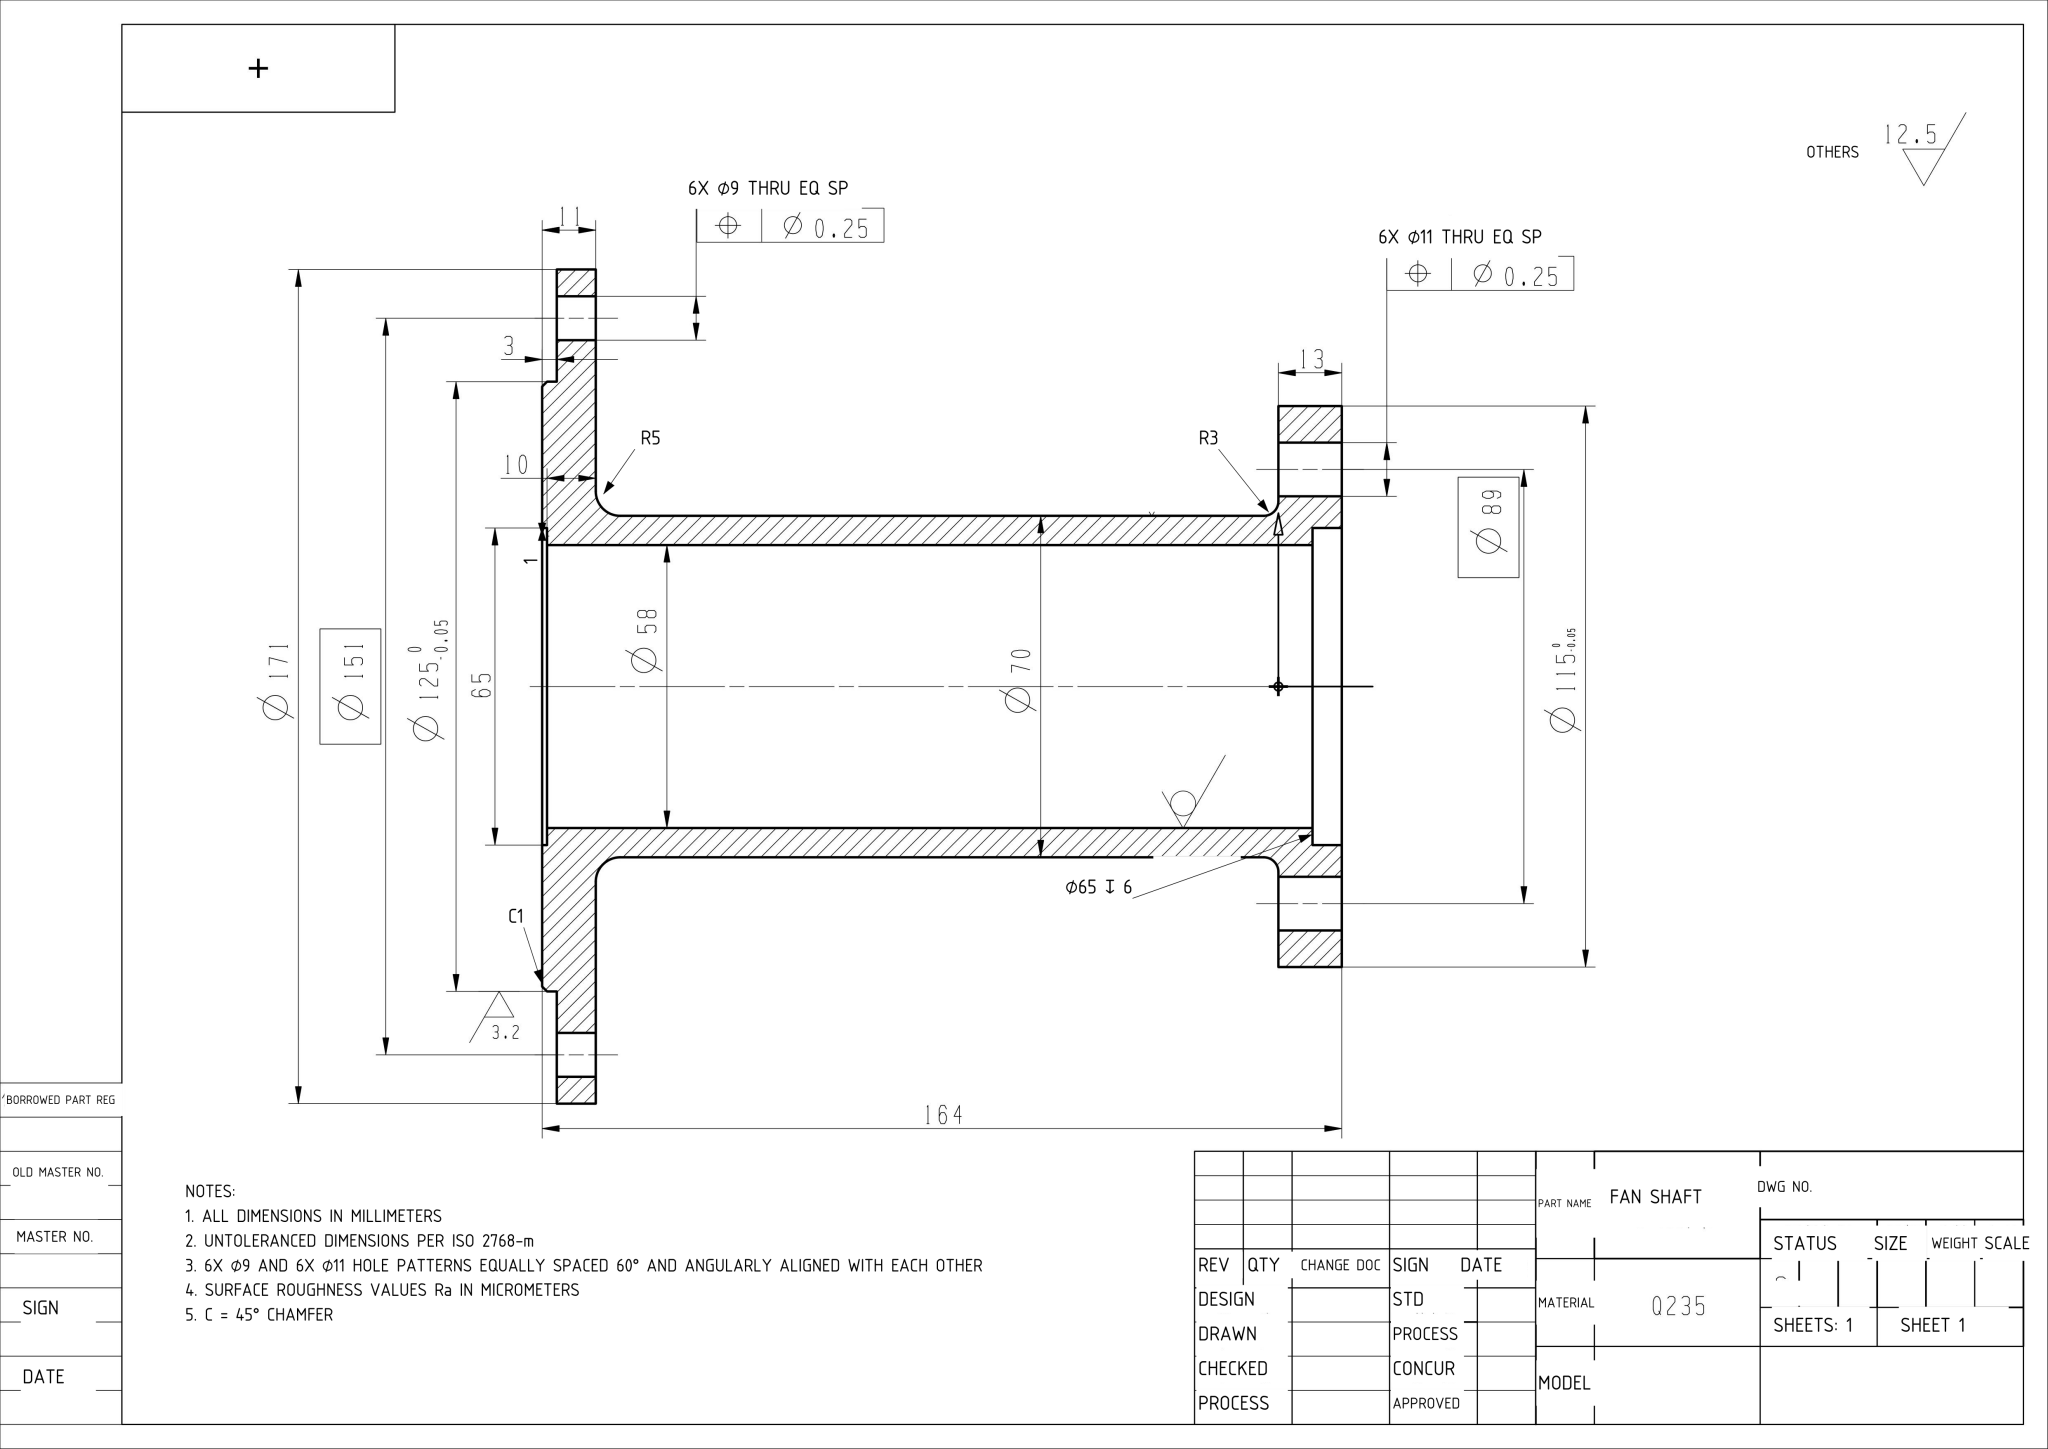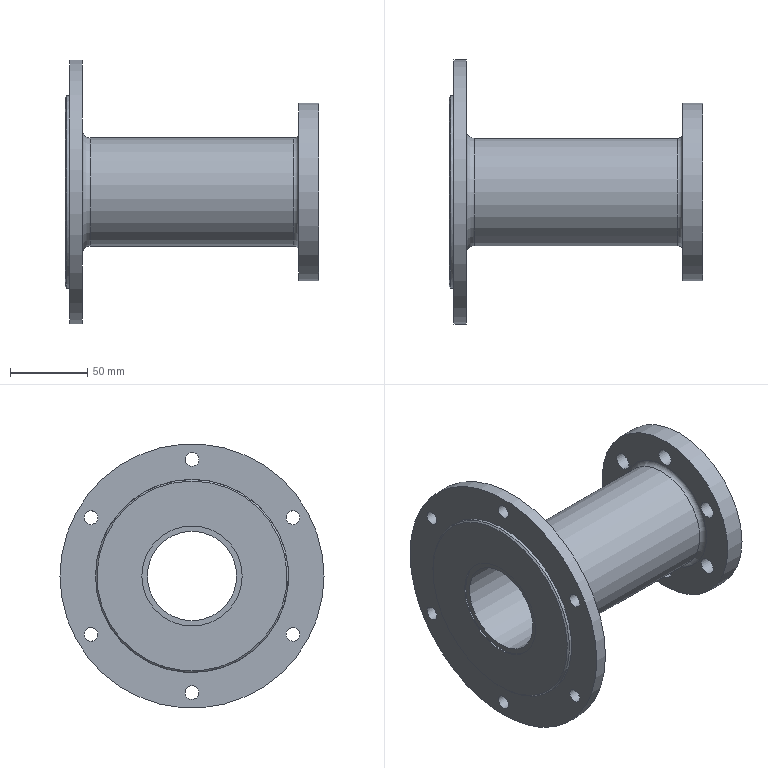Part | NX | mm | 1 solid | 29 faces | box 164 x 171 x 171 mm | volume 447309 mm3 | cylinder 19 | plane 7 | torus 2 | cone 1 | commonest cylinder face diameters 11 x6 9 x6 65 x2 70 x1 58 x1 115 x1 171 x1 125 x1
STEP:
#1=CARTESIAN_POINT('',(0.,0.,0.));
#2=DIRECTION('',(0.,0.,1.));
#3=DIRECTION('',(1.,0.,0.));
#4=AXIS2_PLACEMENT_3D('',#1,#2,#3);
#5=(LENGTH_UNIT()NAMED_UNIT(*)SI_UNIT(.MILLI.,.METRE.));
#6=UNCERTAINTY_MEASURE_WITH_UNIT(LENGTH_MEASURE(0.00002),#5,'','');
#7=(NAMED_UNIT(*)PLANE_ANGLE_UNIT()SI_UNIT($,.RADIAN.));
#8=PLANE_ANGLE_MEASURE_WITH_UNIT(PLANE_ANGLE_MEASURE(0.01745),#7);
#9=DIMENSIONAL_EXPONENTS(0.,0.,0.,0.,0.,0.,0.);
#10=(CONVERSION_BASED_UNIT('',#8)NAMED_UNIT(#9)PLANE_ANGLE_UNIT());
#11=(NAMED_UNIT(*)SI_UNIT($,.STERADIAN.)SOLID_ANGLE_UNIT());
#12=(GEOMETRIC_REPRESENTATION_CONTEXT(3)GLOBAL_UNCERTAINTY_ASSIGNED_CONTEXT((#6))GLOBAL_UNIT_ASSIGNED_CONTEXT((#5,#10,#11))REPRESENTATION_CONTEXT('',''));
#13=SHAPE_REPRESENTATION('',(#4),#12);
#14=CARTESIAN_POINT('',(-135.,0.,35.));
#15=VERTEX_POINT('',#14);
#16=CARTESIAN_POINT('',(-135.,0.,0.));
#17=DIRECTION('',(1.,0.,0.));
#18=DIRECTION('',(0.,0.,1.));
#19=AXIS2_PLACEMENT_3D('',#16,#17,#18);
#20=CIRCLE('',#19,35.);
#21=EDGE_CURVE('',#15,#15,#20,.T.);
#22=ORIENTED_EDGE('',*,*,#21,.T.);
#23=EDGE_LOOP('',(#22));
#24=FACE_BOUND('',#23,.T.);
#25=CARTESIAN_POINT('',(-3.,0.,-35.));
#26=VERTEX_POINT('',#25);
#27=CARTESIAN_POINT('',(-3.,0.,0.));
#28=DIRECTION('',(-1.,0.,0.));
#29=DIRECTION('',(0.,0.,-1.));
#30=AXIS2_PLACEMENT_3D('',#27,#28,#29);
#31=CIRCLE('',#30,35.);
#32=EDGE_CURVE('',#26,#26,#31,.T.);
#33=ORIENTED_EDGE('',*,*,#32,.T.);
#34=EDGE_LOOP('',(#33));
#35=FACE_BOUND('',#34,.T.);
#36=CARTESIAN_POINT('',(-140.,0.,0.));
#37=DIRECTION('',(1.,0.,0.));
#38=DIRECTION('',(0.,0.,-1.));
#39=AXIS2_PLACEMENT_3D('',#36,#37,#38);
#40=CYLINDRICAL_SURFACE('',#39,35.);
#41=ADVANCED_FACE('',(#24,#35),#40,.T.);
#42=CARTESIAN_POINT('',(-150.,0.,-29.));
#43=VERTEX_POINT('',#42);
#44=CARTESIAN_POINT('',(-150.,0.,0.));
#45=DIRECTION('',(-1.,0.,0.));
#46=DIRECTION('',(0.,0.,-1.));
#47=AXIS2_PLACEMENT_3D('',#44,#45,#46);
#48=CIRCLE('',#47,29.);
#49=EDGE_CURVE('',#43,#43,#48,.T.);
#50=ORIENTED_EDGE('',*,*,#49,.F.);
#51=EDGE_LOOP('',(#50));
#52=FACE_BOUND('',#51,.T.);
#53=CARTESIAN_POINT('',(-150.,32.5,-0.));
#54=VERTEX_POINT('',#53);
#55=CARTESIAN_POINT('',(-150.,0.,0.));
#56=DIRECTION('',(1.,0.,0.));
#57=DIRECTION('',(0.,1.,-0.));
#58=AXIS2_PLACEMENT_3D('',#55,#56,#57);
#59=CIRCLE('',#58,32.5);
#60=EDGE_CURVE('',#54,#54,#59,.T.);
#61=ORIENTED_EDGE('',*,*,#60,.F.);
#62=EDGE_LOOP('',(#61));
#63=FACE_BOUND('',#62,.T.);
#64=CARTESIAN_POINT('',(-150.,0.,0.));
#65=DIRECTION('',(1.,0.,0.));
#66=DIRECTION('',(0.,0.,-1.));
#67=AXIS2_PLACEMENT_3D('',#64,#65,#66);
#68=PLANE('',#67);
#69=ADVANCED_FACE('',(#52,#63),#68,.F.);
#70=CARTESIAN_POINT('',(7.,0.,-29.));
#71=VERTEX_POINT('',#70);
#72=CARTESIAN_POINT('',(7.,0.,0.));
#73=DIRECTION('',(-1.,0.,0.));
#74=DIRECTION('',(0.,0.,-1.));
#75=AXIS2_PLACEMENT_3D('',#72,#73,#74);
#76=CIRCLE('',#75,29.);
#77=EDGE_CURVE('',#71,#71,#76,.T.);
#78=ORIENTED_EDGE('',*,*,#77,.T.);
#79=EDGE_LOOP('',(#78));
#80=FACE_BOUND('',#79,.T.);
#81=CARTESIAN_POINT('',(7.,32.5,-0.));
#82=VERTEX_POINT('',#81);
#83=CARTESIAN_POINT('',(7.,0.,0.));
#84=DIRECTION('',(-1.,0.,0.));
#85=DIRECTION('',(0.,1.,-0.));
#86=AXIS2_PLACEMENT_3D('',#83,#84,#85);
#87=CIRCLE('',#86,32.5);
#88=EDGE_CURVE('',#82,#82,#87,.T.);
#89=ORIENTED_EDGE('',*,*,#88,.F.);
#90=EDGE_LOOP('',(#89));
#91=FACE_BOUND('',#90,.T.);
#92=CARTESIAN_POINT('',(7.,0.,0.));
#93=DIRECTION('',(1.,0.,0.));
#94=DIRECTION('',(0.,0.,-1.));
#95=AXIS2_PLACEMENT_3D('',#92,#93,#94);
#96=PLANE('',#95);
#97=ADVANCED_FACE('',(#80,#91),#96,.T.);
#98=ORIENTED_EDGE('',*,*,#77,.F.);
#99=EDGE_LOOP('',(#98));
#100=FACE_BOUND('',#99,.T.);
#101=ORIENTED_EDGE('',*,*,#49,.T.);
#102=EDGE_LOOP('',(#101));
#103=FACE_BOUND('',#102,.T.);
#104=CARTESIAN_POINT('',(-200.,0.,0.));
#105=DIRECTION('',(1.,0.,0.));
#106=DIRECTION('',(0.,0.,-1.));
#107=AXIS2_PLACEMENT_3D('',#104,#105,#106);
#108=CYLINDRICAL_SURFACE('',#107,29.);
#109=ADVANCED_FACE('',(#100,#103),#108,.F.);
#110=CARTESIAN_POINT('',(13.,0.,-32.5));
#111=VERTEX_POINT('',#110);
#112=CARTESIAN_POINT('',(13.,0.,0.));
#113=DIRECTION('',(1.,0.,0.));
#114=DIRECTION('',(0.,0.,-1.));
#115=AXIS2_PLACEMENT_3D('',#112,#113,#114);
#116=CIRCLE('',#115,32.5);
#117=EDGE_CURVE('',#111,#111,#116,.T.);
#118=ORIENTED_EDGE('',*,*,#117,.T.);
#119=EDGE_LOOP('',(#118));
#120=FACE_BOUND('',#119,.T.);
#121=ORIENTED_EDGE('',*,*,#88,.T.);
#122=EDGE_LOOP('',(#121));
#123=FACE_BOUND('',#122,.T.);
#124=CARTESIAN_POINT('',(20.,0.,0.));
#125=DIRECTION('',(-1.,0.,0.));
#126=DIRECTION('',(0.,0.,1.));
#127=AXIS2_PLACEMENT_3D('',#124,#125,#126);
#128=CYLINDRICAL_SURFACE('',#127,32.5);
#129=ADVANCED_FACE('',(#120,#123),#128,.F.);
#130=CARTESIAN_POINT('',(13.,57.5,-0.));
#131=VERTEX_POINT('',#130);
#132=CARTESIAN_POINT('',(13.,0.,0.));
#133=DIRECTION('',(1.,0.,0.));
#134=DIRECTION('',(0.,1.,-0.));
#135=AXIS2_PLACEMENT_3D('',#132,#133,#134);
#136=CIRCLE('',#135,57.5);
#137=EDGE_CURVE('',#131,#131,#136,.T.);
#138=ORIENTED_EDGE('',*,*,#137,.F.);
#139=EDGE_LOOP('',(#138));
#140=FACE_BOUND('',#139,.T.);
#141=CARTESIAN_POINT('',(0.,57.5,-0.));
#142=VERTEX_POINT('',#141);
#143=CARTESIAN_POINT('',(0.,0.,0.));
#144=DIRECTION('',(1.,0.,0.));
#145=DIRECTION('',(0.,1.,-0.));
#146=AXIS2_PLACEMENT_3D('',#143,#144,#145);
#147=CIRCLE('',#146,57.5);
#148=EDGE_CURVE('',#142,#142,#147,.T.);
#149=ORIENTED_EDGE('',*,*,#148,.T.);
#150=EDGE_LOOP('',(#149));
#151=FACE_BOUND('',#150,.T.);
#152=CARTESIAN_POINT('',(13.,0.,0.));
#153=DIRECTION('',(-1.,0.,0.));
#154=DIRECTION('',(0.,0.,1.));
#155=AXIS2_PLACEMENT_3D('',#152,#153,#154);
#156=CYLINDRICAL_SURFACE('',#155,57.5);
#157=ADVANCED_FACE('',(#140,#151),#156,.T.);
#158=CARTESIAN_POINT('',(13.,38.538,16.75));
#159=VERTEX_POINT('',#158);
#160=CARTESIAN_POINT('',(13.,38.538,22.25));
#161=DIRECTION('',(-1.,0.,0.));
#162=DIRECTION('',(0.,0.,-1.));
#163=AXIS2_PLACEMENT_3D('',#160,#161,#162);
#164=CIRCLE('',#163,5.5);
#165=EDGE_CURVE('',#159,#159,#164,.T.);
#166=ORIENTED_EDGE('',*,*,#165,.T.);
#167=EDGE_LOOP('',(#166));
#168=FACE_BOUND('',#167,.T.);
#169=CARTESIAN_POINT('',(13.,38.538,-27.75));
#170=VERTEX_POINT('',#169);
#171=CARTESIAN_POINT('',(13.,38.538,-22.25));
#172=DIRECTION('',(-1.,0.,0.));
#173=DIRECTION('',(0.,0.,-1.));
#174=AXIS2_PLACEMENT_3D('',#171,#172,#173);
#175=CIRCLE('',#174,5.5);
#176=EDGE_CURVE('',#170,#170,#175,.T.);
#177=ORIENTED_EDGE('',*,*,#176,.T.);
#178=EDGE_LOOP('',(#177));
#179=FACE_BOUND('',#178,.T.);
#180=CARTESIAN_POINT('',(13.,-0.,-50.));
#181=VERTEX_POINT('',#180);
#182=CARTESIAN_POINT('',(13.,-0.,-44.5));
#183=DIRECTION('',(-1.,0.,0.));
#184=DIRECTION('',(0.,0.,-1.));
#185=AXIS2_PLACEMENT_3D('',#182,#183,#184);
#186=CIRCLE('',#185,5.5);
#187=EDGE_CURVE('',#181,#181,#186,.T.);
#188=ORIENTED_EDGE('',*,*,#187,.T.);
#189=EDGE_LOOP('',(#188));
#190=FACE_BOUND('',#189,.T.);
#191=CARTESIAN_POINT('',(13.,-38.538,-27.75));
#192=VERTEX_POINT('',#191);
#193=CARTESIAN_POINT('',(13.,-38.538,-22.25));
#194=DIRECTION('',(-1.,0.,0.));
#195=DIRECTION('',(0.,0.,-1.));
#196=AXIS2_PLACEMENT_3D('',#193,#194,#195);
#197=CIRCLE('',#196,5.5);
#198=EDGE_CURVE('',#192,#192,#197,.T.);
#199=ORIENTED_EDGE('',*,*,#198,.T.);
#200=EDGE_LOOP('',(#199));
#201=FACE_BOUND('',#200,.T.);
#202=CARTESIAN_POINT('',(13.,-38.538,16.75));
#203=VERTEX_POINT('',#202);
#204=CARTESIAN_POINT('',(13.,-38.538,22.25));
#205=DIRECTION('',(-1.,0.,0.));
#206=DIRECTION('',(0.,0.,-1.));
#207=AXIS2_PLACEMENT_3D('',#204,#205,#206);
#208=CIRCLE('',#207,5.5);
#209=EDGE_CURVE('',#203,#203,#208,.T.);
#210=ORIENTED_EDGE('',*,*,#209,.T.);
#211=EDGE_LOOP('',(#210));
#212=FACE_BOUND('',#211,.T.);
#213=CARTESIAN_POINT('',(13.,0.,39.));
#214=VERTEX_POINT('',#213);
#215=CARTESIAN_POINT('',(13.,0.,44.5));
#216=DIRECTION('',(-1.,0.,0.));
#217=DIRECTION('',(0.,0.,-1.));
#218=AXIS2_PLACEMENT_3D('',#215,#216,#217);
#219=CIRCLE('',#218,5.5);
#220=EDGE_CURVE('',#214,#214,#219,.T.);
#221=ORIENTED_EDGE('',*,*,#220,.T.);
#222=EDGE_LOOP('',(#221));
#223=FACE_BOUND('',#222,.T.);
#224=ORIENTED_EDGE('',*,*,#117,.F.);
#225=EDGE_LOOP('',(#224));
#226=FACE_BOUND('',#225,.T.);
#227=ORIENTED_EDGE('',*,*,#137,.T.);
#228=EDGE_LOOP('',(#227));
#229=FACE_BOUND('',#228,.T.);
#230=CARTESIAN_POINT('',(13.,0.,0.));
#231=DIRECTION('',(1.,0.,0.));
#232=DIRECTION('',(0.,0.,-1.));
#233=AXIS2_PLACEMENT_3D('',#230,#231,#232);
#234=PLANE('',#233);
#235=ADVANCED_FACE('',(#168,#179,#190,#201,#212,#223,#226,#229),#234,.T.);
#236=CARTESIAN_POINT('',(0.,0.,-38.));
#237=VERTEX_POINT('',#236);
#238=CARTESIAN_POINT('',(0.,0.,0.));
#239=DIRECTION('',(1.,0.,0.));
#240=DIRECTION('',(0.,0.,-1.));
#241=AXIS2_PLACEMENT_3D('',#238,#239,#240);
#242=CIRCLE('',#241,38.);
#243=EDGE_CURVE('',#237,#237,#242,.T.);
#244=ORIENTED_EDGE('',*,*,#243,.T.);
#245=EDGE_LOOP('',(#244));
#246=FACE_BOUND('',#245,.T.);
#247=CARTESIAN_POINT('',(0.,41.288,17.487));
#248=VERTEX_POINT('',#247);
#249=CARTESIAN_POINT('',(0.,38.538,22.25));
#250=DIRECTION('',(1.,0.,0.));
#251=DIRECTION('',(0.,0.5,-0.866));
#252=AXIS2_PLACEMENT_3D('',#249,#250,#251);
#253=CIRCLE('',#252,5.5);
#254=EDGE_CURVE('',#248,#248,#253,.T.);
#255=ORIENTED_EDGE('',*,*,#254,.T.);
#256=EDGE_LOOP('',(#255));
#257=FACE_BOUND('',#256,.T.);
#258=CARTESIAN_POINT('',(0.,35.788,-27.013));
#259=VERTEX_POINT('',#258);
#260=CARTESIAN_POINT('',(0.,38.538,-22.25));
#261=DIRECTION('',(1.,0.,0.));
#262=DIRECTION('',(0.,-0.5,-0.866));
#263=AXIS2_PLACEMENT_3D('',#260,#261,#262);
#264=CIRCLE('',#263,5.5);
#265=EDGE_CURVE('',#259,#259,#264,.T.);
#266=ORIENTED_EDGE('',*,*,#265,.T.);
#267=EDGE_LOOP('',(#266));
#268=FACE_BOUND('',#267,.T.);
#269=CARTESIAN_POINT('',(0.,-5.5,-44.5));
#270=VERTEX_POINT('',#269);
#271=CARTESIAN_POINT('',(0.,-0.,-44.5));
#272=DIRECTION('',(1.,0.,0.));
#273=DIRECTION('',(0.,-1.,0.));
#274=AXIS2_PLACEMENT_3D('',#271,#272,#273);
#275=CIRCLE('',#274,5.5);
#276=EDGE_CURVE('',#270,#270,#275,.T.);
#277=ORIENTED_EDGE('',*,*,#276,.T.);
#278=EDGE_LOOP('',(#277));
#279=FACE_BOUND('',#278,.T.);
#280=CARTESIAN_POINT('',(0.,-41.288,-17.487));
#281=VERTEX_POINT('',#280);
#282=CARTESIAN_POINT('',(0.,-38.538,-22.25));
#283=DIRECTION('',(1.,0.,0.));
#284=DIRECTION('',(0.,-0.5,0.866));
#285=AXIS2_PLACEMENT_3D('',#282,#283,#284);
#286=CIRCLE('',#285,5.5);
#287=EDGE_CURVE('',#281,#281,#286,.T.);
#288=ORIENTED_EDGE('',*,*,#287,.T.);
#289=EDGE_LOOP('',(#288));
#290=FACE_BOUND('',#289,.T.);
#291=CARTESIAN_POINT('',(0.,-35.788,27.013));
#292=VERTEX_POINT('',#291);
#293=CARTESIAN_POINT('',(0.,-38.538,22.25));
#294=DIRECTION('',(1.,0.,0.));
#295=DIRECTION('',(0.,0.5,0.866));
#296=AXIS2_PLACEMENT_3D('',#293,#294,#295);
#297=CIRCLE('',#296,5.5);
#298=EDGE_CURVE('',#292,#292,#297,.T.);
#299=ORIENTED_EDGE('',*,*,#298,.T.);
#300=EDGE_LOOP('',(#299));
#301=FACE_BOUND('',#300,.T.);
#302=CARTESIAN_POINT('',(0.,5.5,44.5));
#303=VERTEX_POINT('',#302);
#304=CARTESIAN_POINT('',(0.,0.,44.5));
#305=DIRECTION('',(1.,0.,0.));
#306=DIRECTION('',(0.,1.,0.));
#307=AXIS2_PLACEMENT_3D('',#304,#305,#306);
#308=CIRCLE('',#307,5.5);
#309=EDGE_CURVE('',#303,#303,#308,.T.);
#310=ORIENTED_EDGE('',*,*,#309,.T.);
#311=EDGE_LOOP('',(#310));
#312=FACE_BOUND('',#311,.T.);
#313=ORIENTED_EDGE('',*,*,#148,.F.);
#314=EDGE_LOOP('',(#313));
#315=FACE_BOUND('',#314,.T.);
#316=CARTESIAN_POINT('',(0.,0.,0.));
#317=DIRECTION('',(1.,0.,0.));
#318=DIRECTION('',(0.,0.,-1.));
#319=AXIS2_PLACEMENT_3D('',#316,#317,#318);
#320=PLANE('',#319);
#321=ADVANCED_FACE('',(#246,#257,#268,#279,#290,#301,#312,#315),#320,.F.);
#322=ORIENTED_EDGE('',*,*,#220,.F.);
#323=EDGE_LOOP('',(#322));
#324=FACE_BOUND('',#323,.T.);
#325=ORIENTED_EDGE('',*,*,#309,.F.);
#326=EDGE_LOOP('',(#325));
#327=FACE_BOUND('',#326,.T.);
#328=CARTESIAN_POINT('',(20.,0.,44.5));
#329=DIRECTION('',(-1.,0.,0.));
#330=DIRECTION('',(0.,0.,1.));
#331=AXIS2_PLACEMENT_3D('',#328,#329,#330);
#332=CYLINDRICAL_SURFACE('',#331,5.5);
#333=ADVANCED_FACE('',(#324,#327),#332,.F.);
#334=ORIENTED_EDGE('',*,*,#209,.F.);
#335=EDGE_LOOP('',(#334));
#336=FACE_BOUND('',#335,.T.);
#337=ORIENTED_EDGE('',*,*,#298,.F.);
#338=EDGE_LOOP('',(#337));
#339=FACE_BOUND('',#338,.T.);
#340=CARTESIAN_POINT('',(20.,-38.538,22.25));
#341=DIRECTION('',(-1.,0.,0.));
#342=DIRECTION('',(0.,0.,1.));
#343=AXIS2_PLACEMENT_3D('',#340,#341,#342);
#344=CYLINDRICAL_SURFACE('',#343,5.5);
#345=ADVANCED_FACE('',(#336,#339),#344,.F.);
#346=ORIENTED_EDGE('',*,*,#198,.F.);
#347=EDGE_LOOP('',(#346));
#348=FACE_BOUND('',#347,.T.);
#349=ORIENTED_EDGE('',*,*,#287,.F.);
#350=EDGE_LOOP('',(#349));
#351=FACE_BOUND('',#350,.T.);
#352=CARTESIAN_POINT('',(20.,-38.538,-22.25));
#353=DIRECTION('',(-1.,0.,0.));
#354=DIRECTION('',(0.,0.,1.));
#355=AXIS2_PLACEMENT_3D('',#352,#353,#354);
#356=CYLINDRICAL_SURFACE('',#355,5.5);
#357=ADVANCED_FACE('',(#348,#351),#356,.F.);
#358=ORIENTED_EDGE('',*,*,#187,.F.);
#359=EDGE_LOOP('',(#358));
#360=FACE_BOUND('',#359,.T.);
#361=ORIENTED_EDGE('',*,*,#276,.F.);
#362=EDGE_LOOP('',(#361));
#363=FACE_BOUND('',#362,.T.);
#364=CARTESIAN_POINT('',(20.,-0.,-44.5));
#365=DIRECTION('',(-1.,0.,0.));
#366=DIRECTION('',(0.,0.,1.));
#367=AXIS2_PLACEMENT_3D('',#364,#365,#366);
#368=CYLINDRICAL_SURFACE('',#367,5.5);
#369=ADVANCED_FACE('',(#360,#363),#368,.F.);
#370=ORIENTED_EDGE('',*,*,#176,.F.);
#371=EDGE_LOOP('',(#370));
#372=FACE_BOUND('',#371,.T.);
#373=ORIENTED_EDGE('',*,*,#265,.F.);
#374=EDGE_LOOP('',(#373));
#375=FACE_BOUND('',#374,.T.);
#376=CARTESIAN_POINT('',(20.,38.538,-22.25));
#377=DIRECTION('',(-1.,0.,0.));
#378=DIRECTION('',(0.,0.,1.));
#379=AXIS2_PLACEMENT_3D('',#376,#377,#378);
#380=CYLINDRICAL_SURFACE('',#379,5.5);
#381=ADVANCED_FACE('',(#372,#375),#380,.F.);
#382=ORIENTED_EDGE('',*,*,#165,.F.);
#383=EDGE_LOOP('',(#382));
#384=FACE_BOUND('',#383,.T.);
#385=ORIENTED_EDGE('',*,*,#254,.F.);
#386=EDGE_LOOP('',(#385));
#387=FACE_BOUND('',#386,.T.);
#388=CARTESIAN_POINT('',(20.,38.538,22.25));
#389=DIRECTION('',(-1.,0.,0.));
#390=DIRECTION('',(0.,0.,1.));
#391=AXIS2_PLACEMENT_3D('',#388,#389,#390);
#392=CYLINDRICAL_SURFACE('',#391,5.5);
#393=ADVANCED_FACE('',(#384,#387),#392,.F.);
#394=CARTESIAN_POINT('',(-140.,0.,40.));
#395=VERTEX_POINT('',#394);
#396=CARTESIAN_POINT('',(-140.,0.,0.));
#397=DIRECTION('',(-1.,0.,0.));
#398=DIRECTION('',(0.,0.,1.));
#399=AXIS2_PLACEMENT_3D('',#396,#397,#398);
#400=CIRCLE('',#399,40.);
#401=EDGE_CURVE('',#395,#395,#400,.T.);
#402=ORIENTED_EDGE('',*,*,#401,.T.);
#403=EDGE_LOOP('',(#402));
#404=FACE_BOUND('',#403,.T.);
#405=CARTESIAN_POINT('',(-140.,85.5,0.));
#406=VERTEX_POINT('',#405);
#407=CARTESIAN_POINT('',(-140.,0.,0.));
#408=DIRECTION('',(-1.,0.,0.));
#409=DIRECTION('',(0.,1.,0.));
#410=AXIS2_PLACEMENT_3D('',#407,#408,#409);
#411=CIRCLE('',#410,85.5);
#412=EDGE_CURVE('',#406,#406,#411,.T.);
#413=ORIENTED_EDGE('',*,*,#412,.F.);
#414=EDGE_LOOP('',(#413));
#415=FACE_BOUND('',#414,.T.);
#416=CARTESIAN_POINT('',(-140.,4.5,-75.5));
#417=VERTEX_POINT('',#416);
#418=CARTESIAN_POINT('',(-140.,0.,-75.5));
#419=DIRECTION('',(1.,0.,0.));
#420=DIRECTION('',(0.,1.,0.));
#421=AXIS2_PLACEMENT_3D('',#418,#419,#420);
#422=CIRCLE('',#421,4.5);
#423=EDGE_CURVE('',#417,#417,#422,.T.);
#424=ORIENTED_EDGE('',*,*,#423,.F.);
#425=EDGE_LOOP('',(#424));
#426=FACE_BOUND('',#425,.T.);
#427=CARTESIAN_POINT('',(-140.,67.635,-33.853));
#428=VERTEX_POINT('',#427);
#429=CARTESIAN_POINT('',(-140.,65.385,-37.75));
#430=DIRECTION('',(1.,0.,0.));
#431=DIRECTION('',(0.,0.5,0.866));
#432=AXIS2_PLACEMENT_3D('',#429,#430,#431);
#433=CIRCLE('',#432,4.5);
#434=EDGE_CURVE('',#428,#428,#433,.T.);
#435=ORIENTED_EDGE('',*,*,#434,.F.);
#436=EDGE_LOOP('',(#435));
#437=FACE_BOUND('',#436,.T.);
#438=CARTESIAN_POINT('',(-140.,63.135,41.647));
#439=VERTEX_POINT('',#438);
#440=CARTESIAN_POINT('',(-140.,65.385,37.75));
#441=DIRECTION('',(1.,0.,0.));
#442=DIRECTION('',(0.,-0.5,0.866));
#443=AXIS2_PLACEMENT_3D('',#440,#441,#442);
#444=CIRCLE('',#443,4.5);
#445=EDGE_CURVE('',#439,#439,#444,.T.);
#446=ORIENTED_EDGE('',*,*,#445,.F.);
#447=EDGE_LOOP('',(#446));
#448=FACE_BOUND('',#447,.T.);
#449=CARTESIAN_POINT('',(-140.,-4.5,75.5));
#450=VERTEX_POINT('',#449);
#451=CARTESIAN_POINT('',(-140.,0.,75.5));
#452=DIRECTION('',(1.,0.,0.));
#453=DIRECTION('',(0.,-1.,0.));
#454=AXIS2_PLACEMENT_3D('',#451,#452,#453);
#455=CIRCLE('',#454,4.5);
#456=EDGE_CURVE('',#450,#450,#455,.T.);
#457=ORIENTED_EDGE('',*,*,#456,.F.);
#458=EDGE_LOOP('',(#457));
#459=FACE_BOUND('',#458,.T.);
#460=CARTESIAN_POINT('',(-140.,-67.635,33.853));
#461=VERTEX_POINT('',#460);
#462=CARTESIAN_POINT('',(-140.,-65.385,37.75));
#463=DIRECTION('',(1.,0.,0.));
#464=DIRECTION('',(0.,-0.5,-0.866));
#465=AXIS2_PLACEMENT_3D('',#462,#463,#464);
#466=CIRCLE('',#465,4.5);
#467=EDGE_CURVE('',#461,#461,#466,.T.);
#468=ORIENTED_EDGE('',*,*,#467,.F.);
#469=EDGE_LOOP('',(#468));
#470=FACE_BOUND('',#469,.T.);
#471=CARTESIAN_POINT('',(-140.,-63.135,-41.647));
#472=VERTEX_POINT('',#471);
#473=CARTESIAN_POINT('',(-140.,-65.385,-37.75));
#474=DIRECTION('',(1.,0.,0.));
#475=DIRECTION('',(0.,0.5,-0.866));
#476=AXIS2_PLACEMENT_3D('',#473,#474,#475);
#477=CIRCLE('',#476,4.5);
#478=EDGE_CURVE('',#472,#472,#477,.T.);
#479=ORIENTED_EDGE('',*,*,#478,.F.);
#480=EDGE_LOOP('',(#479));
#481=FACE_BOUND('',#480,.T.);
#482=CARTESIAN_POINT('',(-140.,0.,0.));
#483=DIRECTION('',(-1.,0.,0.));
#484=DIRECTION('',(0.,0.,1.));
#485=AXIS2_PLACEMENT_3D('',#482,#483,#484);
#486=PLANE('',#485);
#487=ADVANCED_FACE('',(#404,#415,#426,#437,#448,#459,#470,#481),#486,.F.);
#488=ORIENTED_EDGE('',*,*,#412,.T.);
#489=EDGE_LOOP('',(#488));
#490=FACE_BOUND('',#489,.T.);
#491=CARTESIAN_POINT('',(-148.,85.5,0.));
#492=VERTEX_POINT('',#491);
#493=CARTESIAN_POINT('',(-148.,0.,0.));
#494=DIRECTION('',(-1.,0.,0.));
#495=DIRECTION('',(0.,1.,0.));
#496=AXIS2_PLACEMENT_3D('',#493,#494,#495);
#497=CIRCLE('',#496,85.5);
#498=EDGE_CURVE('',#492,#492,#497,.T.);
#499=ORIENTED_EDGE('',*,*,#498,.F.);
#500=EDGE_LOOP('',(#499));
#501=FACE_BOUND('',#500,.T.);
#502=CARTESIAN_POINT('',(-151.,0.,0.));
#503=DIRECTION('',(1.,0.,0.));
#504=DIRECTION('',(0.,0.,-1.));
#505=AXIS2_PLACEMENT_3D('',#502,#503,#504);
#506=CYLINDRICAL_SURFACE('',#505,85.5);
#507=ADVANCED_FACE('',(#490,#501),#506,.T.);
#508=CARTESIAN_POINT('',(-151.,0.,61.5));
#509=VERTEX_POINT('',#508);
#510=CARTESIAN_POINT('',(-151.,0.,0.));
#511=DIRECTION('',(-1.,0.,0.));
#512=DIRECTION('',(0.,0.,1.));
#513=AXIS2_PLACEMENT_3D('',#510,#511,#512);
#514=CIRCLE('',#513,61.5);
#515=EDGE_CURVE('',#509,#509,#514,.T.);
#516=ORIENTED_EDGE('',*,*,#515,.T.);
#517=EDGE_LOOP('',(#516));
#518=FACE_BOUND('',#517,.T.);
#519=CARTESIAN_POINT('',(-151.,32.5,0.));
#520=VERTEX_POINT('',#519);
#521=CARTESIAN_POINT('',(-151.,0.,0.));
#522=DIRECTION('',(-1.,0.,0.));
#523=DIRECTION('',(0.,1.,0.));
#524=AXIS2_PLACEMENT_3D('',#521,#522,#523);
#525=CIRCLE('',#524,32.5);
#526=EDGE_CURVE('',#520,#520,#525,.T.);
#527=ORIENTED_EDGE('',*,*,#526,.F.);
#528=EDGE_LOOP('',(#527));
#529=FACE_BOUND('',#528,.T.);
#530=CARTESIAN_POINT('',(-151.,0.,0.));
#531=DIRECTION('',(-1.,0.,0.));
#532=DIRECTION('',(0.,0.,1.));
#533=AXIS2_PLACEMENT_3D('',#530,#531,#532);
#534=PLANE('',#533);
#535=ADVANCED_FACE('',(#518,#529),#534,.T.);
#536=ORIENTED_EDGE('',*,*,#60,.T.);
#537=EDGE_LOOP('',(#536));
#538=FACE_BOUND('',#537,.T.);
#539=ORIENTED_EDGE('',*,*,#526,.T.);
#540=EDGE_LOOP('',(#539));
#541=FACE_BOUND('',#540,.T.);
#542=CARTESIAN_POINT('',(-151.,0.,0.));
#543=DIRECTION('',(1.,0.,0.));
#544=DIRECTION('',(0.,0.,-1.));
#545=AXIS2_PLACEMENT_3D('',#542,#543,#544);
#546=CYLINDRICAL_SURFACE('',#545,32.5);
#547=ADVANCED_FACE('',(#538,#541),#546,.F.);
#548=CARTESIAN_POINT('',(-150.,0.,62.5));
#549=VERTEX_POINT('',#548);
#550=CARTESIAN_POINT('',(-150.,0.,0.));
#551=DIRECTION('',(1.,0.,0.));
#552=DIRECTION('',(0.,0.,1.));
#553=AXIS2_PLACEMENT_3D('',#550,#551,#552);
#554=CIRCLE('',#553,62.5);
#555=EDGE_CURVE('',#549,#549,#554,.T.);
#556=ORIENTED_EDGE('',*,*,#555,.T.);
#557=EDGE_LOOP('',(#556));
#558=FACE_BOUND('',#557,.T.);
#559=CARTESIAN_POINT('',(-148.,62.5,0.));
#560=VERTEX_POINT('',#559);
#561=CARTESIAN_POINT('',(-148.,0.,0.));
#562=DIRECTION('',(-1.,0.,0.));
#563=DIRECTION('',(0.,1.,0.));
#564=AXIS2_PLACEMENT_3D('',#561,#562,#563);
#565=CIRCLE('',#564,62.5);
#566=EDGE_CURVE('',#560,#560,#565,.T.);
#567=ORIENTED_EDGE('',*,*,#566,.T.);
#568=EDGE_LOOP('',(#567));
#569=FACE_BOUND('',#568,.T.);
#570=CARTESIAN_POINT('',(-151.,0.,0.));
#571=DIRECTION('',(1.,0.,0.));
#572=DIRECTION('',(0.,0.,-1.));
#573=AXIS2_PLACEMENT_3D('',#570,#571,#572);
#574=CYLINDRICAL_SURFACE('',#573,62.5);
#575=ADVANCED_FACE('',(#558,#569),#574,.T.);
#576=CARTESIAN_POINT('',(-148.,-65.385,-33.25));
#577=VERTEX_POINT('',#576);
#578=CARTESIAN_POINT('',(-148.,-65.385,-37.75));
#579=DIRECTION('',(-1.,0.,0.));
#580=DIRECTION('',(0.,0.,1.));
#581=AXIS2_PLACEMENT_3D('',#578,#579,#580);
#582=CIRCLE('',#581,4.5);
#583=EDGE_CURVE('',#577,#577,#582,.T.);
#584=ORIENTED_EDGE('',*,*,#583,.F.);
#585=EDGE_LOOP('',(#584));
#586=FACE_BOUND('',#585,.T.);
#587=CARTESIAN_POINT('',(-148.,-65.385,42.25));
#588=VERTEX_POINT('',#587);
#589=CARTESIAN_POINT('',(-148.,-65.385,37.75));
#590=DIRECTION('',(-1.,0.,0.));
#591=DIRECTION('',(0.,0.,1.));
#592=AXIS2_PLACEMENT_3D('',#589,#590,#591);
#593=CIRCLE('',#592,4.5);
#594=EDGE_CURVE('',#588,#588,#593,.T.);
#595=ORIENTED_EDGE('',*,*,#594,.F.);
#596=EDGE_LOOP('',(#595));
#597=FACE_BOUND('',#596,.T.);
#598=CARTESIAN_POINT('',(-148.,0.,80.));
#599=VERTEX_POINT('',#598);
#600=CARTESIAN_POINT('',(-148.,0.,75.5));
#601=DIRECTION('',(-1.,0.,0.));
#602=DIRECTION('',(0.,0.,1.));
#603=AXIS2_PLACEMENT_3D('',#600,#601,#602);
#604=CIRCLE('',#603,4.5);
#605=EDGE_CURVE('',#599,#599,#604,.T.);
#606=ORIENTED_EDGE('',*,*,#605,.F.);
#607=EDGE_LOOP('',(#606));
#608=FACE_BOUND('',#607,.T.);
#609=CARTESIAN_POINT('',(-148.,65.385,42.25));
#610=VERTEX_POINT('',#609);
#611=CARTESIAN_POINT('',(-148.,65.385,37.75));
#612=DIRECTION('',(-1.,0.,0.));
#613=DIRECTION('',(0.,0.,1.));
#614=AXIS2_PLACEMENT_3D('',#611,#612,#613);
#615=CIRCLE('',#614,4.5);
#616=EDGE_CURVE('',#610,#610,#615,.T.);
#617=ORIENTED_EDGE('',*,*,#616,.F.);
#618=EDGE_LOOP('',(#617));
#619=FACE_BOUND('',#618,.T.);
#620=CARTESIAN_POINT('',(-148.,65.385,-33.25));
#621=VERTEX_POINT('',#620);
#622=CARTESIAN_POINT('',(-148.,65.385,-37.75));
#623=DIRECTION('',(-1.,0.,0.));
#624=DIRECTION('',(0.,0.,1.));
#625=AXIS2_PLACEMENT_3D('',#622,#623,#624);
#626=CIRCLE('',#625,4.5);
#627=EDGE_CURVE('',#621,#621,#626,.T.);
#628=ORIENTED_EDGE('',*,*,#627,.F.);
#629=EDGE_LOOP('',(#628));
#630=FACE_BOUND('',#629,.T.);
#631=CARTESIAN_POINT('',(-148.,0.,-71.));
#632=VERTEX_POINT('',#631);
#633=CARTESIAN_POINT('',(-148.,0.,-75.5));
#634=DIRECTION('',(-1.,0.,0.));
#635=DIRECTION('',(0.,0.,1.));
#636=AXIS2_PLACEMENT_3D('',#633,#634,#635);
#637=CIRCLE('',#636,4.5);
#638=EDGE_CURVE('',#632,#632,#637,.T.);
#639=ORIENTED_EDGE('',*,*,#638,.F.);
#640=EDGE_LOOP('',(#639));
#641=FACE_BOUND('',#640,.T.);
#642=ORIENTED_EDGE('',*,*,#498,.T.);
#643=EDGE_LOOP('',(#642));
#644=FACE_BOUND('',#643,.T.);
#645=ORIENTED_EDGE('',*,*,#566,.F.);
#646=EDGE_LOOP('',(#645));
#647=FACE_BOUND('',#646,.T.);
#648=CARTESIAN_POINT('',(-148.,0.,0.));
#649=DIRECTION('',(-1.,0.,0.));
#650=DIRECTION('',(0.,0.,1.));
#651=AXIS2_PLACEMENT_3D('',#648,#649,#650);
#652=PLANE('',#651);
#653=ADVANCED_FACE('',(#586,#597,#608,#619,#630,#641,#644,#647),#652,.T.);
#654=ORIENTED_EDGE('',*,*,#515,.F.);
#655=EDGE_LOOP('',(#654));
#656=FACE_BOUND('',#655,.T.);
#657=ORIENTED_EDGE('',*,*,#555,.F.);
#658=EDGE_LOOP('',(#657));
#659=FACE_BOUND('',#658,.T.);
#660=CARTESIAN_POINT('',(-150.,0.,0.));
#661=DIRECTION('',(1.,0.,0.));
#662=DIRECTION('',(0.,0.,-1.));
#663=AXIS2_PLACEMENT_3D('',#660,#661,#662);
#664=CONICAL_SURFACE('',#663,62.5,45.);
#665=ADVANCED_FACE('',(#656,#659),#664,.T.);
#666=ORIENTED_EDGE('',*,*,#638,.T.);
#667=EDGE_LOOP('',(#666));
#668=FACE_BOUND('',#667,.T.);
#669=ORIENTED_EDGE('',*,*,#423,.T.);
#670=EDGE_LOOP('',(#669));
#671=FACE_BOUND('',#670,.T.);
#672=CARTESIAN_POINT('',(-160.,0.,-75.5));
#673=DIRECTION('',(1.,0.,0.));
#674=DIRECTION('',(0.,0.,-1.));
#675=AXIS2_PLACEMENT_3D('',#672,#673,#674);
#676=CYLINDRICAL_SURFACE('',#675,4.5);
#677=ADVANCED_FACE('',(#668,#671),#676,.F.);
#678=ORIENTED_EDGE('',*,*,#627,.T.);
#679=EDGE_LOOP('',(#678));
#680=FACE_BOUND('',#679,.T.);
#681=ORIENTED_EDGE('',*,*,#434,.T.);
#682=EDGE_LOOP('',(#681));
#683=FACE_BOUND('',#682,.T.);
#684=CARTESIAN_POINT('',(-160.,65.385,-37.75));
#685=DIRECTION('',(1.,0.,0.));
#686=DIRECTION('',(0.,0.,-1.));
#687=AXIS2_PLACEMENT_3D('',#684,#685,#686);
#688=CYLINDRICAL_SURFACE('',#687,4.5);
#689=ADVANCED_FACE('',(#680,#683),#688,.F.);
#690=ORIENTED_EDGE('',*,*,#616,.T.);
#691=EDGE_LOOP('',(#690));
#692=FACE_BOUND('',#691,.T.);
#693=ORIENTED_EDGE('',*,*,#445,.T.);
#694=EDGE_LOOP('',(#693));
#695=FACE_BOUND('',#694,.T.);
#696=CARTESIAN_POINT('',(-160.,65.385,37.75));
#697=DIRECTION('',(1.,0.,0.));
#698=DIRECTION('',(0.,0.,-1.));
#699=AXIS2_PLACEMENT_3D('',#696,#697,#698);
#700=CYLINDRICAL_SURFACE('',#699,4.5);
#701=ADVANCED_FACE('',(#692,#695),#700,.F.);
#702=ORIENTED_EDGE('',*,*,#605,.T.);
#703=EDGE_LOOP('',(#702));
#704=FACE_BOUND('',#703,.T.);
#705=ORIENTED_EDGE('',*,*,#456,.T.);
#706=EDGE_LOOP('',(#705));
#707=FACE_BOUND('',#706,.T.);
#708=CARTESIAN_POINT('',(-160.,0.,75.5));
#709=DIRECTION('',(1.,0.,0.));
#710=DIRECTION('',(0.,0.,-1.));
#711=AXIS2_PLACEMENT_3D('',#708,#709,#710);
#712=CYLINDRICAL_SURFACE('',#711,4.5);
#713=ADVANCED_FACE('',(#704,#707),#712,.F.);
#714=ORIENTED_EDGE('',*,*,#594,.T.);
#715=EDGE_LOOP('',(#714));
#716=FACE_BOUND('',#715,.T.);
#717=ORIENTED_EDGE('',*,*,#467,.T.);
#718=EDGE_LOOP('',(#717));
#719=FACE_BOUND('',#718,.T.);
#720=CARTESIAN_POINT('',(-160.,-65.385,37.75));
#721=DIRECTION('',(1.,0.,0.));
#722=DIRECTION('',(0.,0.,-1.));
#723=AXIS2_PLACEMENT_3D('',#720,#721,#722);
#724=CYLINDRICAL_SURFACE('',#723,4.5);
#725=ADVANCED_FACE('',(#716,#719),#724,.F.);
#726=ORIENTED_EDGE('',*,*,#583,.T.);
#727=EDGE_LOOP('',(#726));
#728=FACE_BOUND('',#727,.T.);
#729=ORIENTED_EDGE('',*,*,#478,.T.);
#730=EDGE_LOOP('',(#729));
#731=FACE_BOUND('',#730,.T.);
#732=CARTESIAN_POINT('',(-160.,-65.385,-37.75));
#733=DIRECTION('',(1.,0.,0.));
#734=DIRECTION('',(0.,0.,-1.));
#735=AXIS2_PLACEMENT_3D('',#732,#733,#734);
#736=CYLINDRICAL_SURFACE('',#735,4.5);
#737=ADVANCED_FACE('',(#728,#731),#736,.F.);
#738=ORIENTED_EDGE('',*,*,#243,.F.);
#739=EDGE_LOOP('',(#738));
#740=FACE_BOUND('',#739,.T.);
#741=ORIENTED_EDGE('',*,*,#32,.F.);
#742=EDGE_LOOP('',(#741));
#743=FACE_BOUND('',#742,.T.);
#744=CARTESIAN_POINT('',(-3.,0.,0.));
#745=DIRECTION('',(1.,0.,0.));
#746=DIRECTION('',(0.,0.,-1.));
#747=AXIS2_PLACEMENT_3D('',#744,#745,#746);
#748=TOROIDAL_SURFACE('',#747,38.,3.);
#749=ADVANCED_FACE('',(#740,#743),#748,.F.);
#750=ORIENTED_EDGE('',*,*,#21,.F.);
#751=EDGE_LOOP('',(#750));
#752=FACE_BOUND('',#751,.T.);
#753=ORIENTED_EDGE('',*,*,#401,.F.);
#754=EDGE_LOOP('',(#753));
#755=FACE_BOUND('',#754,.T.);
#756=CARTESIAN_POINT('',(-135.,0.,0.));
#757=DIRECTION('',(-1.,0.,0.));
#758=DIRECTION('',(0.,0.,1.));
#759=AXIS2_PLACEMENT_3D('',#756,#757,#758);
#760=TOROIDAL_SURFACE('',#759,40.,5.);
#761=ADVANCED_FACE('',(#752,#755),#760,.F.);
#762=CLOSED_SHELL('',(#41,#69,#97,#109,#129,#157,#235,#321,#333,#345,#357,#369,#381,#393,#487,#507,#535,#547,#575,#653,#665,#677,#689,#701,#713,#725,#737,#749,#761));
#763=MANIFOLD_SOLID_BREP('',#762);
#764=ADVANCED_BREP_SHAPE_REPRESENTATION('',(#763),#12);
#765=SHAPE_REPRESENTATION_RELATIONSHIP('','',#13,#764);
#766=PRESENTATION_LAYER_ASSIGNMENT('','',(#763));
#767=COLOUR_RGB('',1.,0.6,0.);
#768=FILL_AREA_STYLE_COLOUR('',#767);
#769=FILL_AREA_STYLE('',(#768));
#770=SURFACE_STYLE_FILL_AREA(#769);
#771=SURFACE_SIDE_STYLE('',(#770));
#772=SURFACE_STYLE_USAGE(.BOTH.,#771);
#773=PRESENTATION_STYLE_ASSIGNMENT((#772));
#774=STYLED_ITEM('',(#773),#763);
#775=MECHANICAL_DESIGN_GEOMETRIC_PRESENTATION_REPRESENTATION('',(#774),#12);